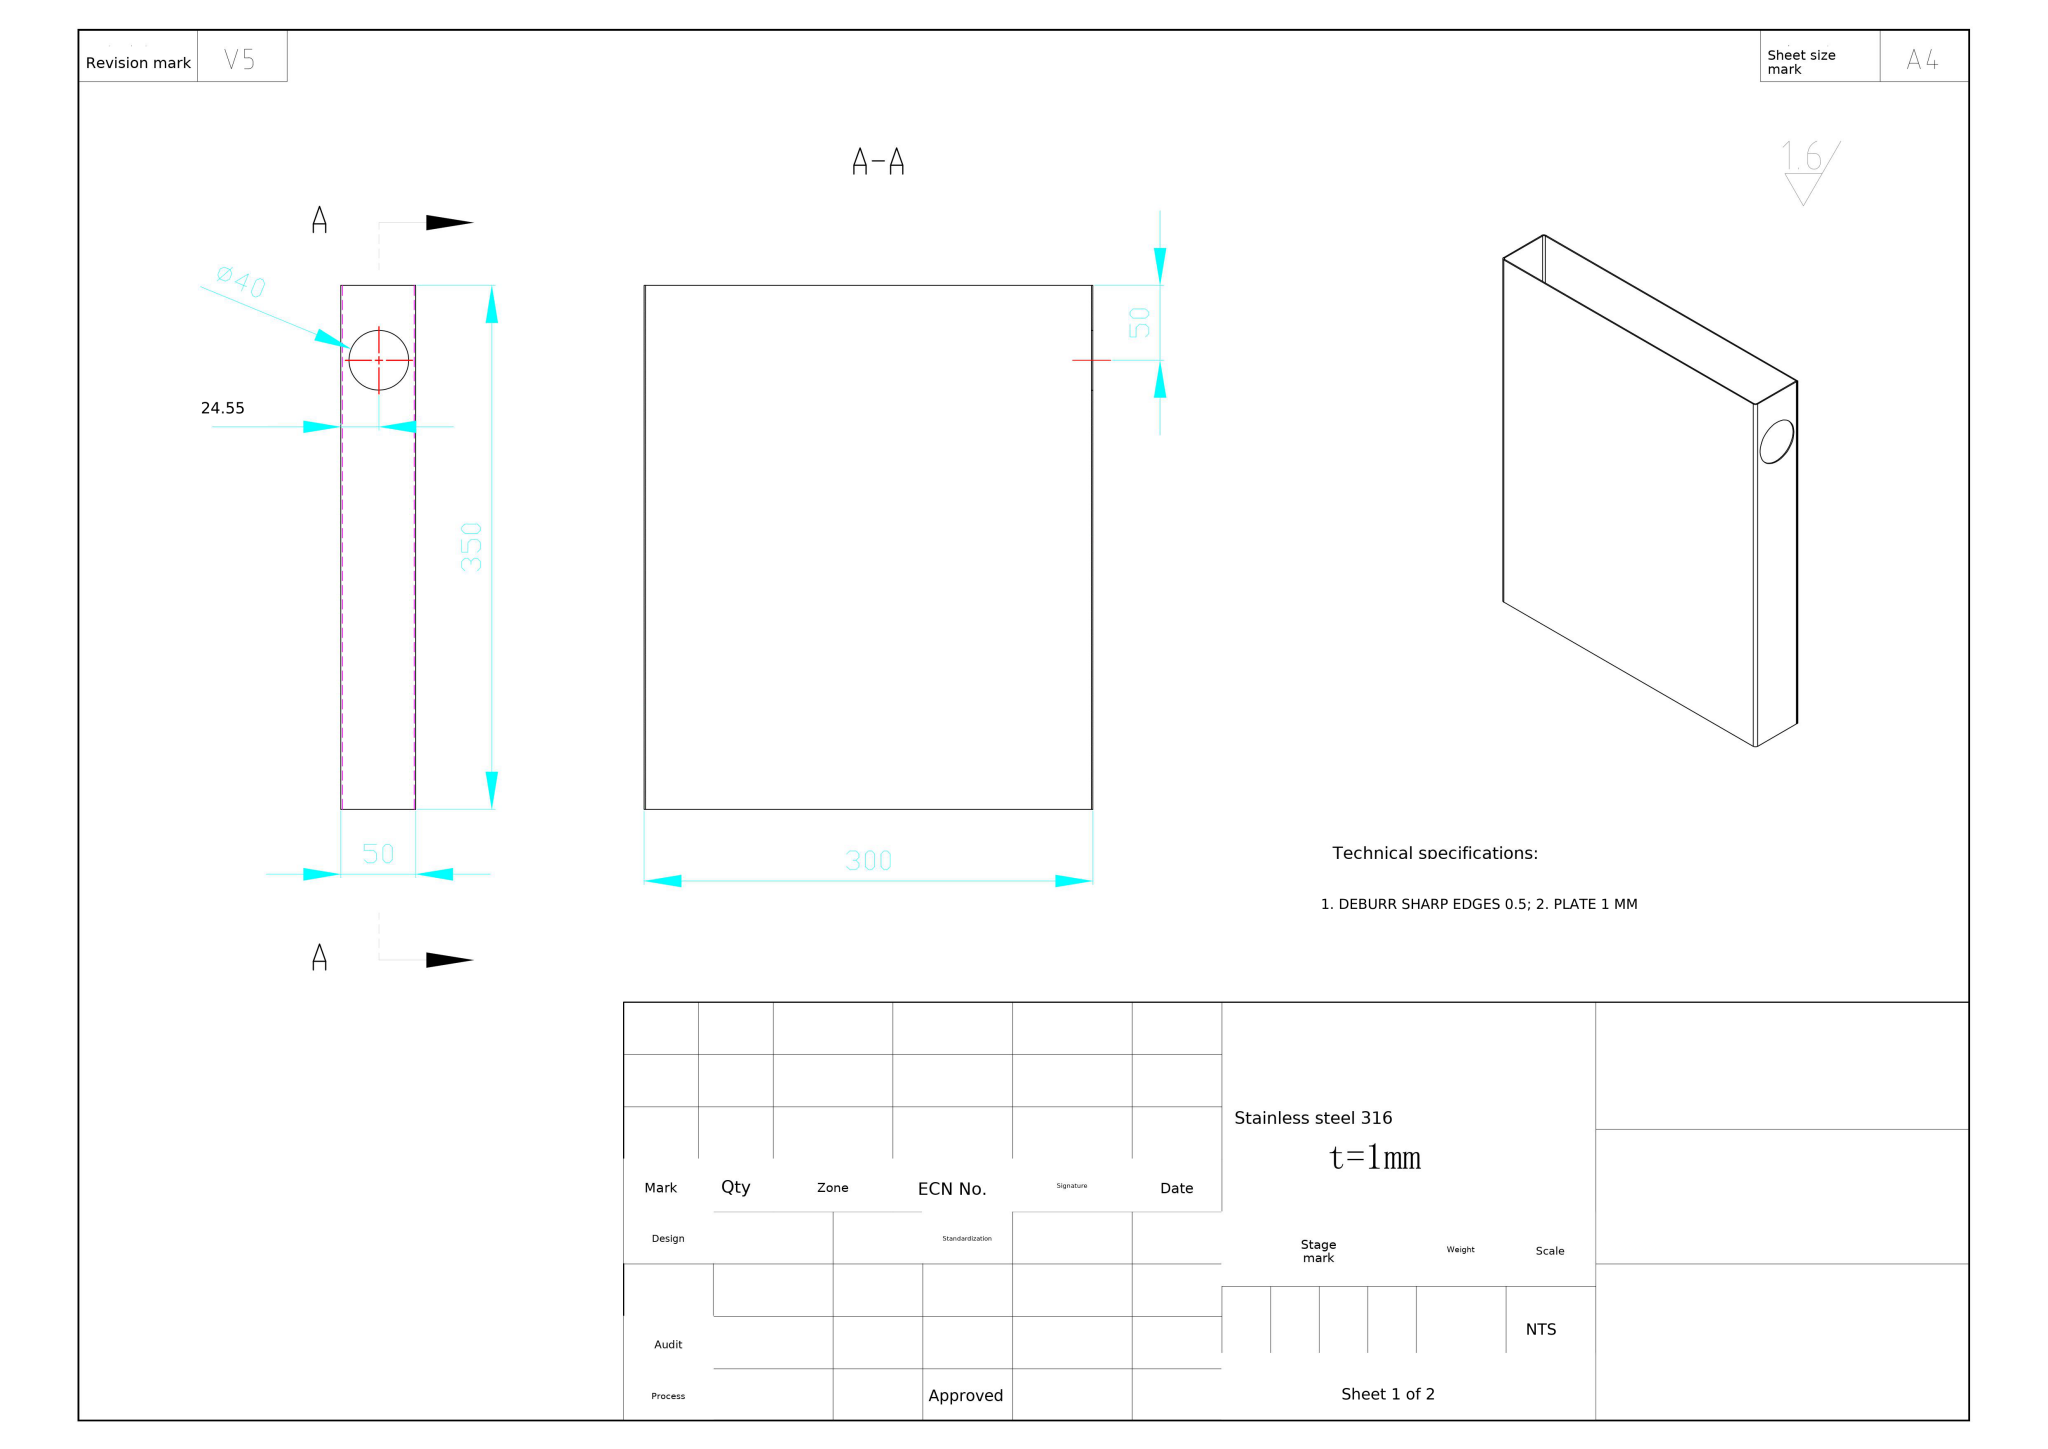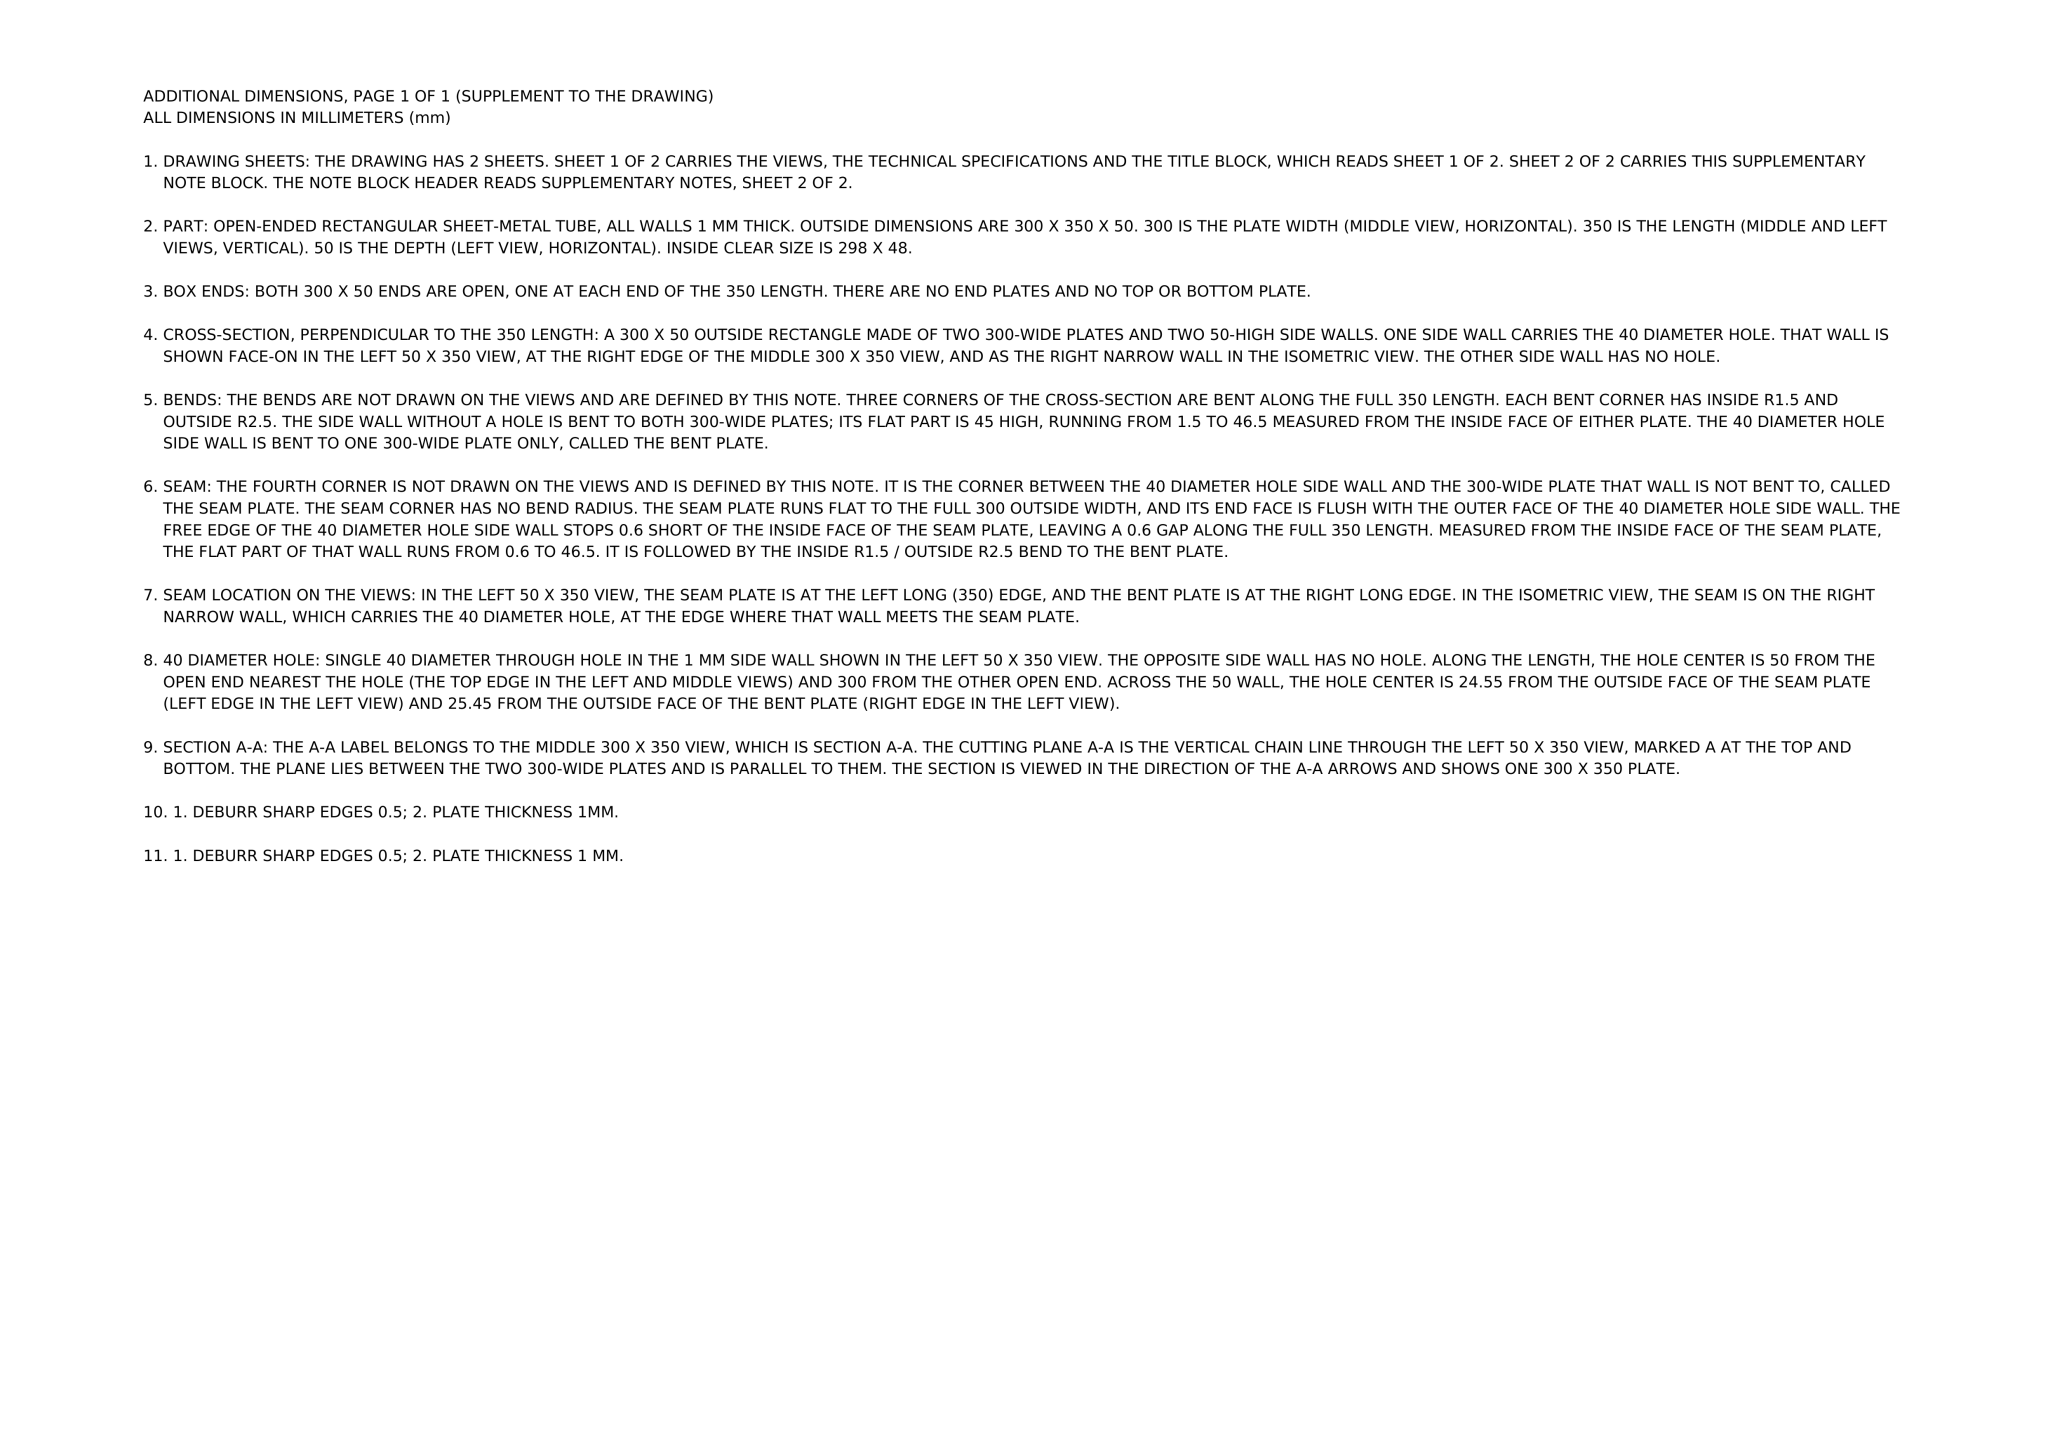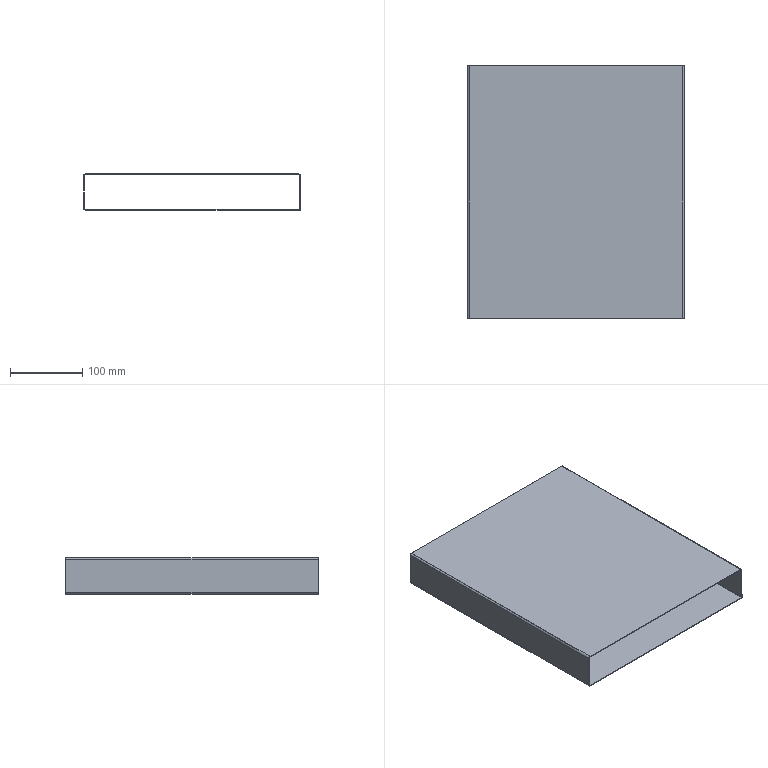Part | NX | mm | 1 solid | 32 faces | box 300 x 350 x 50 mm | volume 241232 mm3 | plane 24 | cylinder 8 | commonest cylinder face diameters 5 x3 3 x3 40 x2